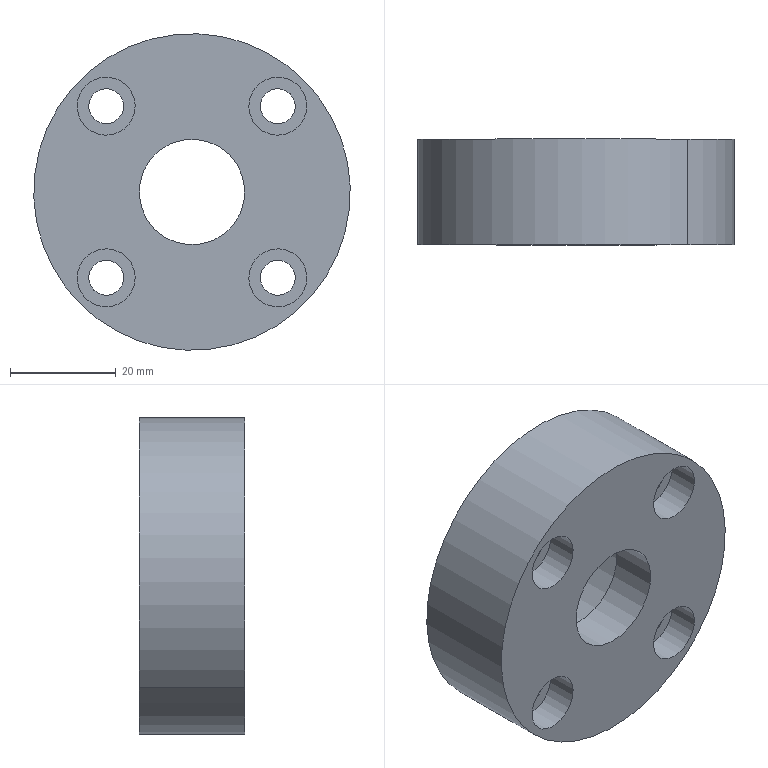Component | SolidWorks | LowerRollerFixingRing-5 | 1 solid | 29 faces | box 60 x 20 x 60 mm | volume 38941 mm3 | cylinder 22 | plane 7 | commonest cylinder face diameters 11 x8 6.6 x8 20 x2 35 x2 60 x2
STEP:
#1=COLOUR_RGB('',0.7922,0.8196,0.9333);
#2=FILL_AREA_STYLE_COLOUR('',#1);
#3=FILL_AREA_STYLE('',(#2));
#4=SURFACE_STYLE_FILL_AREA(#3);
#5=SURFACE_SIDE_STYLE('',(#4));
#6=SURFACE_STYLE_USAGE(.BOTH.,#5);
#7=PRESENTATION_STYLE_ASSIGNMENT((#6));
#8=CARTESIAN_POINT('',(-5.128,20.59,-6.45));
#9=VERTEX_POINT('',#8);
#10=CARTESIAN_POINT('',(-4.822,20.59,-6.144));
#11=VERTEX_POINT('',#10);
#12=CARTESIAN_POINT('',(-4.975,20.59,-6.297));
#13=DIRECTION('',(0.,-1.,-0.));
#14=DIRECTION('',(0.7071,0.,0.7071));
#15=AXIS2_PLACEMENT_3D('',#12,#13,#14);
#16=CIRCLE('',#15,0.2165);
#17=EDGE_CURVE('',#9,#11,#16,.T.);
#18=ORIENTED_EDGE('',*,*,#17,.F.);
#19=CARTESIAN_POINT('',(-5.128,20.354,-6.45));
#20=VERTEX_POINT('',#19);
#21=CARTESIAN_POINT('',(-5.128,20.354,-6.45));
#22=DIRECTION('',(0.,-1.,-0.));
#23=VECTOR('',#22,39.37);
#24=LINE('',#21,#23);
#25=EDGE_CURVE('',#9,#20,#24,.T.);
#26=ORIENTED_EDGE('',*,*,#25,.T.);
#27=CARTESIAN_POINT('',(-4.822,20.354,-6.144));
#28=VERTEX_POINT('',#27);
#29=CARTESIAN_POINT('',(-4.975,20.354,-6.297));
#30=DIRECTION('',(0.,-1.,-0.));
#31=DIRECTION('',(0.7071,0.,0.7071));
#32=AXIS2_PLACEMENT_3D('',#29,#30,#31);
#33=CIRCLE('',#32,0.2165);
#34=EDGE_CURVE('',#20,#28,#33,.T.);
#35=ORIENTED_EDGE('',*,*,#34,.T.);
#36=CARTESIAN_POINT('',(-4.822,20.354,-6.144));
#37=DIRECTION('',(0.,-1.,-0.));
#38=VECTOR('',#37,39.37);
#39=LINE('',#36,#38);
#40=EDGE_CURVE('',#11,#28,#39,.T.);
#41=ORIENTED_EDGE('',*,*,#40,.F.);
#42=EDGE_LOOP('',(#18,#26,#35,#41));
#43=FACE_OUTER_BOUND('',#42,.T.);
#44=CARTESIAN_POINT('',(-4.975,20.354,-6.297));
#45=DIRECTION('',(0.,-1.,-0.));
#46=DIRECTION('',(0.7071,0.,0.7071));
#47=AXIS2_PLACEMENT_3D('',#44,#45,#46);
#48=CYLINDRICAL_SURFACE('',#47,0.2165);
#49=ADVANCED_FACE('',(#43),#48,.F.);
#50=CARTESIAN_POINT('',(-5.067,21.141,-6.389));
#51=VERTEX_POINT('',#50);
#52=CARTESIAN_POINT('',(-4.883,21.141,-6.205));
#53=VERTEX_POINT('',#52);
#54=CARTESIAN_POINT('',(-4.975,21.141,-6.297));
#55=DIRECTION('',(0.,-1.,-0.));
#56=DIRECTION('',(0.7071,0.,0.7071));
#57=AXIS2_PLACEMENT_3D('',#54,#55,#56);
#58=CIRCLE('',#57,0.1299);
#59=EDGE_CURVE('',#51,#53,#58,.T.);
#60=ORIENTED_EDGE('',*,*,#59,.F.);
#61=CARTESIAN_POINT('',(-5.067,20.59,-6.389));
#62=VERTEX_POINT('',#61);
#63=CARTESIAN_POINT('',(-5.067,20.354,-6.389));
#64=DIRECTION('',(0.,-1.,-0.));
#65=VECTOR('',#64,39.37);
#66=LINE('',#63,#65);
#67=EDGE_CURVE('',#51,#62,#66,.T.);
#68=ORIENTED_EDGE('',*,*,#67,.T.);
#69=CARTESIAN_POINT('',(-4.883,20.59,-6.205));
#70=VERTEX_POINT('',#69);
#71=CARTESIAN_POINT('',(-4.975,20.59,-6.297));
#72=DIRECTION('',(0.,-1.,-0.));
#73=DIRECTION('',(0.7071,0.,0.7071));
#74=AXIS2_PLACEMENT_3D('',#71,#72,#73);
#75=CIRCLE('',#74,0.1299);
#76=EDGE_CURVE('',#62,#70,#75,.T.);
#77=ORIENTED_EDGE('',*,*,#76,.T.);
#78=CARTESIAN_POINT('',(-4.883,20.354,-6.205));
#79=DIRECTION('',(0.,-1.,-0.));
#80=VECTOR('',#79,39.37);
#81=LINE('',#78,#80);
#82=EDGE_CURVE('',#53,#70,#81,.T.);
#83=ORIENTED_EDGE('',*,*,#82,.F.);
#84=EDGE_LOOP('',(#60,#68,#77,#83));
#85=FACE_OUTER_BOUND('',#84,.T.);
#86=CARTESIAN_POINT('',(-4.975,20.354,-6.297));
#87=DIRECTION('',(0.,-1.,-0.));
#88=DIRECTION('',(0.7071,0.,0.7071));
#89=AXIS2_PLACEMENT_3D('',#86,#87,#88);
#90=CYLINDRICAL_SURFACE('',#89,0.1299);
#91=ADVANCED_FACE('',(#85),#90,.F.);
#92=CARTESIAN_POINT('',(-5.128,20.59,-7.731));
#93=VERTEX_POINT('',#92);
#94=CARTESIAN_POINT('',(-4.822,20.59,-7.425));
#95=VERTEX_POINT('',#94);
#96=CARTESIAN_POINT('',(-4.975,20.59,-7.578));
#97=DIRECTION('',(0.,-1.,-0.));
#98=DIRECTION('',(0.7071,0.,0.7071));
#99=AXIS2_PLACEMENT_3D('',#96,#97,#98);
#100=CIRCLE('',#99,0.2165);
#101=EDGE_CURVE('',#93,#95,#100,.T.);
#102=ORIENTED_EDGE('',*,*,#101,.F.);
#103=CARTESIAN_POINT('',(-5.128,20.354,-7.731));
#104=VERTEX_POINT('',#103);
#105=CARTESIAN_POINT('',(-5.128,20.354,-7.731));
#106=DIRECTION('',(0.,-1.,-0.));
#107=VECTOR('',#106,39.37);
#108=LINE('',#105,#107);
#109=EDGE_CURVE('',#93,#104,#108,.T.);
#110=ORIENTED_EDGE('',*,*,#109,.T.);
#111=CARTESIAN_POINT('',(-4.822,20.354,-7.425));
#112=VERTEX_POINT('',#111);
#113=CARTESIAN_POINT('',(-4.975,20.354,-7.578));
#114=DIRECTION('',(0.,-1.,-0.));
#115=DIRECTION('',(0.7071,0.,0.7071));
#116=AXIS2_PLACEMENT_3D('',#113,#114,#115);
#117=CIRCLE('',#116,0.2165);
#118=EDGE_CURVE('',#104,#112,#117,.T.);
#119=ORIENTED_EDGE('',*,*,#118,.T.);
#120=CARTESIAN_POINT('',(-4.822,20.354,-7.425));
#121=DIRECTION('',(0.,-1.,-0.));
#122=VECTOR('',#121,39.37);
#123=LINE('',#120,#122);
#124=EDGE_CURVE('',#95,#112,#123,.T.);
#125=ORIENTED_EDGE('',*,*,#124,.F.);
#126=EDGE_LOOP('',(#102,#110,#119,#125));
#127=FACE_OUTER_BOUND('',#126,.T.);
#128=CARTESIAN_POINT('',(-4.975,20.354,-7.578));
#129=DIRECTION('',(0.,-1.,-0.));
#130=DIRECTION('',(0.7071,0.,0.7071));
#131=AXIS2_PLACEMENT_3D('',#128,#129,#130);
#132=CYLINDRICAL_SURFACE('',#131,0.2165);
#133=ADVANCED_FACE('',(#127),#132,.F.);
#134=CARTESIAN_POINT('',(-5.067,21.141,-7.67));
#135=VERTEX_POINT('',#134);
#136=CARTESIAN_POINT('',(-4.883,21.141,-7.486));
#137=VERTEX_POINT('',#136);
#138=CARTESIAN_POINT('',(-4.975,21.141,-7.578));
#139=DIRECTION('',(0.,-1.,-0.));
#140=DIRECTION('',(0.7071,0.,0.7071));
#141=AXIS2_PLACEMENT_3D('',#138,#139,#140);
#142=CIRCLE('',#141,0.1299);
#143=EDGE_CURVE('',#135,#137,#142,.T.);
#144=ORIENTED_EDGE('',*,*,#143,.F.);
#145=CARTESIAN_POINT('',(-5.067,20.59,-7.67));
#146=VERTEX_POINT('',#145);
#147=CARTESIAN_POINT('',(-5.067,20.354,-7.67));
#148=DIRECTION('',(0.,-1.,-0.));
#149=VECTOR('',#148,39.37);
#150=LINE('',#147,#149);
#151=EDGE_CURVE('',#135,#146,#150,.T.);
#152=ORIENTED_EDGE('',*,*,#151,.T.);
#153=CARTESIAN_POINT('',(-4.883,20.59,-7.486));
#154=VERTEX_POINT('',#153);
#155=CARTESIAN_POINT('',(-4.975,20.59,-7.578));
#156=DIRECTION('',(0.,-1.,-0.));
#157=DIRECTION('',(0.7071,0.,0.7071));
#158=AXIS2_PLACEMENT_3D('',#155,#156,#157);
#159=CIRCLE('',#158,0.1299);
#160=EDGE_CURVE('',#146,#154,#159,.T.);
#161=ORIENTED_EDGE('',*,*,#160,.T.);
#162=CARTESIAN_POINT('',(-4.883,20.354,-7.486));
#163=DIRECTION('',(0.,-1.,-0.));
#164=VECTOR('',#163,39.37);
#165=LINE('',#162,#164);
#166=EDGE_CURVE('',#137,#154,#165,.T.);
#167=ORIENTED_EDGE('',*,*,#166,.F.);
#168=EDGE_LOOP('',(#144,#152,#161,#167));
#169=FACE_OUTER_BOUND('',#168,.T.);
#170=CARTESIAN_POINT('',(-4.975,20.354,-7.578));
#171=DIRECTION('',(0.,-1.,-0.));
#172=DIRECTION('',(0.7071,0.,0.7071));
#173=AXIS2_PLACEMENT_3D('',#170,#171,#172);
#174=CYLINDRICAL_SURFACE('',#173,0.1299);
#175=ADVANCED_FACE('',(#169),#174,.F.);
#176=CARTESIAN_POINT('',(-6.408,20.59,-6.45));
#177=VERTEX_POINT('',#176);
#178=CARTESIAN_POINT('',(-6.102,20.59,-6.144));
#179=VERTEX_POINT('',#178);
#180=CARTESIAN_POINT('',(-6.255,20.59,-6.297));
#181=DIRECTION('',(0.,-1.,-0.));
#182=DIRECTION('',(0.7071,0.,0.7071));
#183=AXIS2_PLACEMENT_3D('',#180,#181,#182);
#184=CIRCLE('',#183,0.2165);
#185=EDGE_CURVE('',#177,#179,#184,.T.);
#186=ORIENTED_EDGE('',*,*,#185,.F.);
#187=CARTESIAN_POINT('',(-6.408,20.354,-6.45));
#188=VERTEX_POINT('',#187);
#189=CARTESIAN_POINT('',(-6.408,20.354,-6.45));
#190=DIRECTION('',(0.,-1.,-0.));
#191=VECTOR('',#190,39.37);
#192=LINE('',#189,#191);
#193=EDGE_CURVE('',#177,#188,#192,.T.);
#194=ORIENTED_EDGE('',*,*,#193,.T.);
#195=CARTESIAN_POINT('',(-6.102,20.354,-6.144));
#196=VERTEX_POINT('',#195);
#197=CARTESIAN_POINT('',(-6.255,20.354,-6.297));
#198=DIRECTION('',(0.,-1.,-0.));
#199=DIRECTION('',(0.7071,0.,0.7071));
#200=AXIS2_PLACEMENT_3D('',#197,#198,#199);
#201=CIRCLE('',#200,0.2165);
#202=EDGE_CURVE('',#188,#196,#201,.T.);
#203=ORIENTED_EDGE('',*,*,#202,.T.);
#204=CARTESIAN_POINT('',(-6.102,20.354,-6.144));
#205=DIRECTION('',(0.,-1.,-0.));
#206=VECTOR('',#205,39.37);
#207=LINE('',#204,#206);
#208=EDGE_CURVE('',#179,#196,#207,.T.);
#209=ORIENTED_EDGE('',*,*,#208,.F.);
#210=EDGE_LOOP('',(#186,#194,#203,#209));
#211=FACE_OUTER_BOUND('',#210,.T.);
#212=CARTESIAN_POINT('',(-6.255,20.354,-6.297));
#213=DIRECTION('',(0.,-1.,-0.));
#214=DIRECTION('',(0.7071,0.,0.7071));
#215=AXIS2_PLACEMENT_3D('',#212,#213,#214);
#216=CYLINDRICAL_SURFACE('',#215,0.2165);
#217=ADVANCED_FACE('',(#211),#216,.F.);
#218=CARTESIAN_POINT('',(-6.347,21.141,-6.389));
#219=VERTEX_POINT('',#218);
#220=CARTESIAN_POINT('',(-6.163,21.141,-6.205));
#221=VERTEX_POINT('',#220);
#222=CARTESIAN_POINT('',(-6.255,21.141,-6.297));
#223=DIRECTION('',(0.,-1.,-0.));
#224=DIRECTION('',(0.7071,0.,0.7071));
#225=AXIS2_PLACEMENT_3D('',#222,#223,#224);
#226=CIRCLE('',#225,0.1299);
#227=EDGE_CURVE('',#219,#221,#226,.T.);
#228=ORIENTED_EDGE('',*,*,#227,.F.);
#229=CARTESIAN_POINT('',(-6.347,20.59,-6.389));
#230=VERTEX_POINT('',#229);
#231=CARTESIAN_POINT('',(-6.347,20.354,-6.389));
#232=DIRECTION('',(0.,-1.,-0.));
#233=VECTOR('',#232,39.37);
#234=LINE('',#231,#233);
#235=EDGE_CURVE('',#219,#230,#234,.T.);
#236=ORIENTED_EDGE('',*,*,#235,.T.);
#237=CARTESIAN_POINT('',(-6.163,20.59,-6.205));
#238=VERTEX_POINT('',#237);
#239=CARTESIAN_POINT('',(-6.255,20.59,-6.297));
#240=DIRECTION('',(0.,-1.,-0.));
#241=DIRECTION('',(0.7071,0.,0.7071));
#242=AXIS2_PLACEMENT_3D('',#239,#240,#241);
#243=CIRCLE('',#242,0.1299);
#244=EDGE_CURVE('',#230,#238,#243,.T.);
#245=ORIENTED_EDGE('',*,*,#244,.T.);
#246=CARTESIAN_POINT('',(-6.163,20.354,-6.205));
#247=DIRECTION('',(0.,-1.,-0.));
#248=VECTOR('',#247,39.37);
#249=LINE('',#246,#248);
#250=EDGE_CURVE('',#221,#238,#249,.T.);
#251=ORIENTED_EDGE('',*,*,#250,.F.);
#252=EDGE_LOOP('',(#228,#236,#245,#251));
#253=FACE_OUTER_BOUND('',#252,.T.);
#254=CARTESIAN_POINT('',(-6.255,20.354,-6.297));
#255=DIRECTION('',(0.,-1.,-0.));
#256=DIRECTION('',(0.7071,0.,0.7071));
#257=AXIS2_PLACEMENT_3D('',#254,#255,#256);
#258=CYLINDRICAL_SURFACE('',#257,0.1299);
#259=ADVANCED_FACE('',(#253),#258,.F.);
#260=CARTESIAN_POINT('',(-6.408,20.59,-7.731));
#261=VERTEX_POINT('',#260);
#262=CARTESIAN_POINT('',(-6.102,20.59,-7.425));
#263=VERTEX_POINT('',#262);
#264=CARTESIAN_POINT('',(-6.255,20.59,-7.578));
#265=DIRECTION('',(0.,-1.,-0.));
#266=DIRECTION('',(0.7071,0.,0.7071));
#267=AXIS2_PLACEMENT_3D('',#264,#265,#266);
#268=CIRCLE('',#267,0.2165);
#269=EDGE_CURVE('',#261,#263,#268,.T.);
#270=ORIENTED_EDGE('',*,*,#269,.F.);
#271=CARTESIAN_POINT('',(-6.408,20.354,-7.731));
#272=VERTEX_POINT('',#271);
#273=CARTESIAN_POINT('',(-6.408,20.354,-7.731));
#274=DIRECTION('',(0.,-1.,-0.));
#275=VECTOR('',#274,39.37);
#276=LINE('',#273,#275);
#277=EDGE_CURVE('',#261,#272,#276,.T.);
#278=ORIENTED_EDGE('',*,*,#277,.T.);
#279=CARTESIAN_POINT('',(-6.102,20.354,-7.425));
#280=VERTEX_POINT('',#279);
#281=CARTESIAN_POINT('',(-6.255,20.354,-7.578));
#282=DIRECTION('',(0.,-1.,-0.));
#283=DIRECTION('',(0.7071,0.,0.7071));
#284=AXIS2_PLACEMENT_3D('',#281,#282,#283);
#285=CIRCLE('',#284,0.2165);
#286=EDGE_CURVE('',#272,#280,#285,.T.);
#287=ORIENTED_EDGE('',*,*,#286,.T.);
#288=CARTESIAN_POINT('',(-6.102,20.354,-7.425));
#289=DIRECTION('',(0.,-1.,-0.));
#290=VECTOR('',#289,39.37);
#291=LINE('',#288,#290);
#292=EDGE_CURVE('',#263,#280,#291,.T.);
#293=ORIENTED_EDGE('',*,*,#292,.F.);
#294=EDGE_LOOP('',(#270,#278,#287,#293));
#295=FACE_OUTER_BOUND('',#294,.T.);
#296=CARTESIAN_POINT('',(-6.255,20.354,-7.578));
#297=DIRECTION('',(0.,-1.,-0.));
#298=DIRECTION('',(0.7071,0.,0.7071));
#299=AXIS2_PLACEMENT_3D('',#296,#297,#298);
#300=CYLINDRICAL_SURFACE('',#299,0.2165);
#301=ADVANCED_FACE('',(#295),#300,.F.);
#302=CARTESIAN_POINT('',(-6.347,21.141,-7.67));
#303=VERTEX_POINT('',#302);
#304=CARTESIAN_POINT('',(-6.163,21.141,-7.486));
#305=VERTEX_POINT('',#304);
#306=CARTESIAN_POINT('',(-6.255,21.141,-7.578));
#307=DIRECTION('',(0.,-1.,-0.));
#308=DIRECTION('',(0.7071,0.,0.7071));
#309=AXIS2_PLACEMENT_3D('',#306,#307,#308);
#310=CIRCLE('',#309,0.1299);
#311=EDGE_CURVE('',#303,#305,#310,.T.);
#312=ORIENTED_EDGE('',*,*,#311,.F.);
#313=CARTESIAN_POINT('',(-6.347,20.59,-7.67));
#314=VERTEX_POINT('',#313);
#315=CARTESIAN_POINT('',(-6.347,20.354,-7.67));
#316=DIRECTION('',(0.,-1.,-0.));
#317=VECTOR('',#316,39.37);
#318=LINE('',#315,#317);
#319=EDGE_CURVE('',#303,#314,#318,.T.);
#320=ORIENTED_EDGE('',*,*,#319,.T.);
#321=CARTESIAN_POINT('',(-6.163,20.59,-7.486));
#322=VERTEX_POINT('',#321);
#323=CARTESIAN_POINT('',(-6.255,20.59,-7.578));
#324=DIRECTION('',(0.,-1.,-0.));
#325=DIRECTION('',(0.7071,0.,0.7071));
#326=AXIS2_PLACEMENT_3D('',#323,#324,#325);
#327=CIRCLE('',#326,0.1299);
#328=EDGE_CURVE('',#314,#322,#327,.T.);
#329=ORIENTED_EDGE('',*,*,#328,.T.);
#330=CARTESIAN_POINT('',(-6.163,20.354,-7.486));
#331=DIRECTION('',(0.,-1.,-0.));
#332=VECTOR('',#331,39.37);
#333=LINE('',#330,#332);
#334=EDGE_CURVE('',#305,#322,#333,.T.);
#335=ORIENTED_EDGE('',*,*,#334,.F.);
#336=EDGE_LOOP('',(#312,#320,#329,#335));
#337=FACE_OUTER_BOUND('',#336,.T.);
#338=CARTESIAN_POINT('',(-6.255,20.354,-7.578));
#339=DIRECTION('',(0.,-1.,-0.));
#340=DIRECTION('',(0.7071,0.,0.7071));
#341=AXIS2_PLACEMENT_3D('',#338,#339,#340);
#342=CYLINDRICAL_SURFACE('',#341,0.1299);
#343=ADVANCED_FACE('',(#337),#342,.F.);
#344=CARTESIAN_POINT('',(-5.337,20.354,-6.659));
#345=VERTEX_POINT('',#344);
#346=CARTESIAN_POINT('',(-5.893,20.354,-7.216));
#347=VERTEX_POINT('',#346);
#348=CARTESIAN_POINT('',(-5.615,20.354,-6.938));
#349=DIRECTION('',(-0.,1.,0.));
#350=DIRECTION('',(-0.7071,0.,-0.7071));
#351=AXIS2_PLACEMENT_3D('',#348,#349,#350);
#352=CIRCLE('',#351,0.3937);
#353=EDGE_CURVE('',#345,#347,#352,.T.);
#354=ORIENTED_EDGE('',*,*,#353,.F.);
#355=CARTESIAN_POINT('',(-5.337,20.708,-6.659));
#356=VERTEX_POINT('',#355);
#357=CARTESIAN_POINT('',(-5.337,21.359,-6.659));
#358=DIRECTION('',(-0.,1.,0.));
#359=VECTOR('',#358,39.37);
#360=LINE('',#357,#359);
#361=EDGE_CURVE('',#345,#356,#360,.T.);
#362=ORIENTED_EDGE('',*,*,#361,.T.);
#363=CARTESIAN_POINT('',(-5.893,20.708,-7.216));
#364=VERTEX_POINT('',#363);
#365=CARTESIAN_POINT('',(-5.615,20.708,-6.938));
#366=DIRECTION('',(-0.,1.,0.));
#367=DIRECTION('',(-0.7071,0.,-0.7071));
#368=AXIS2_PLACEMENT_3D('',#365,#366,#367);
#369=CIRCLE('',#368,0.3937);
#370=EDGE_CURVE('',#356,#364,#369,.T.);
#371=ORIENTED_EDGE('',*,*,#370,.T.);
#372=CARTESIAN_POINT('',(-5.893,21.359,-7.216));
#373=DIRECTION('',(-0.,1.,0.));
#374=VECTOR('',#373,39.37);
#375=LINE('',#372,#374);
#376=EDGE_CURVE('',#347,#364,#375,.T.);
#377=ORIENTED_EDGE('',*,*,#376,.F.);
#378=EDGE_LOOP('',(#354,#362,#371,#377));
#379=FACE_OUTER_BOUND('',#378,.T.);
#380=CARTESIAN_POINT('',(-5.615,21.359,-6.938));
#381=DIRECTION('',(-0.,1.,0.));
#382=DIRECTION('',(-0.7071,0.,-0.7071));
#383=AXIS2_PLACEMENT_3D('',#380,#381,#382);
#384=CYLINDRICAL_SURFACE('',#383,0.3937);
#385=ADVANCED_FACE('',(#379),#384,.F.);
#386=CARTESIAN_POINT('',(-5.128,20.708,-6.45));
#387=VERTEX_POINT('',#386);
#388=CARTESIAN_POINT('',(-6.102,20.708,-7.425));
#389=VERTEX_POINT('',#388);
#390=CARTESIAN_POINT('',(-5.615,20.708,-6.938));
#391=DIRECTION('',(-0.,1.,0.));
#392=DIRECTION('',(-0.7071,0.,-0.7071));
#393=AXIS2_PLACEMENT_3D('',#390,#391,#392);
#394=CIRCLE('',#393,0.689);
#395=EDGE_CURVE('',#387,#389,#394,.T.);
#396=ORIENTED_EDGE('',*,*,#395,.F.);
#397=CARTESIAN_POINT('',(-5.128,21.141,-6.45));
#398=VERTEX_POINT('',#397);
#399=CARTESIAN_POINT('',(-5.128,21.359,-6.45));
#400=DIRECTION('',(-0.,1.,0.));
#401=VECTOR('',#400,39.37);
#402=LINE('',#399,#401);
#403=EDGE_CURVE('',#387,#398,#402,.T.);
#404=ORIENTED_EDGE('',*,*,#403,.T.);
#405=CARTESIAN_POINT('',(-6.102,21.141,-7.425));
#406=VERTEX_POINT('',#405);
#407=CARTESIAN_POINT('',(-5.615,21.141,-6.938));
#408=DIRECTION('',(-0.,1.,0.));
#409=DIRECTION('',(-0.7071,0.,-0.7071));
#410=AXIS2_PLACEMENT_3D('',#407,#408,#409);
#411=CIRCLE('',#410,0.689);
#412=EDGE_CURVE('',#398,#406,#411,.T.);
#413=ORIENTED_EDGE('',*,*,#412,.T.);
#414=CARTESIAN_POINT('',(-6.102,21.359,-7.425));
#415=DIRECTION('',(-0.,1.,0.));
#416=VECTOR('',#415,39.37);
#417=LINE('',#414,#416);
#418=EDGE_CURVE('',#389,#406,#417,.T.);
#419=ORIENTED_EDGE('',*,*,#418,.F.);
#420=EDGE_LOOP('',(#396,#404,#413,#419));
#421=FACE_OUTER_BOUND('',#420,.T.);
#422=CARTESIAN_POINT('',(-5.615,21.359,-6.938));
#423=DIRECTION('',(-0.,1.,0.));
#424=DIRECTION('',(-0.7071,0.,-0.7071));
#425=AXIS2_PLACEMENT_3D('',#422,#423,#424);
#426=CYLINDRICAL_SURFACE('',#425,0.689);
#427=ADVANCED_FACE('',(#421),#426,.F.);
#428=CARTESIAN_POINT('',(-6.45,20.354,-7.773));
#429=VERTEX_POINT('',#428);
#430=CARTESIAN_POINT('',(-4.78,20.354,-6.102));
#431=VERTEX_POINT('',#430);
#432=CARTESIAN_POINT('',(-5.615,20.354,-6.938));
#433=DIRECTION('',(-0.,1.,0.));
#434=DIRECTION('',(-0.7071,0.,-0.7071));
#435=AXIS2_PLACEMENT_3D('',#432,#433,#434);
#436=CIRCLE('',#435,1.181);
#437=EDGE_CURVE('',#429,#431,#436,.T.);
#438=ORIENTED_EDGE('',*,*,#437,.T.);
#439=CARTESIAN_POINT('',(-4.78,21.141,-6.102));
#440=VERTEX_POINT('',#439);
#441=CARTESIAN_POINT('',(-4.78,21.359,-6.102));
#442=DIRECTION('',(-0.,1.,0.));
#443=VECTOR('',#442,39.37);
#444=LINE('',#441,#443);
#445=EDGE_CURVE('',#431,#440,#444,.T.);
#446=ORIENTED_EDGE('',*,*,#445,.T.);
#447=CARTESIAN_POINT('',(-6.45,21.141,-7.773));
#448=VERTEX_POINT('',#447);
#449=CARTESIAN_POINT('',(-5.615,21.141,-6.938));
#450=DIRECTION('',(-0.,1.,0.));
#451=DIRECTION('',(-0.7071,0.,-0.7071));
#452=AXIS2_PLACEMENT_3D('',#449,#450,#451);
#453=CIRCLE('',#452,1.181);
#454=EDGE_CURVE('',#448,#440,#453,.T.);
#455=ORIENTED_EDGE('',*,*,#454,.F.);
#456=CARTESIAN_POINT('',(-6.45,21.359,-7.773));
#457=DIRECTION('',(-0.,1.,0.));
#458=VECTOR('',#457,39.37);
#459=LINE('',#456,#458);
#460=EDGE_CURVE('',#429,#448,#459,.T.);
#461=ORIENTED_EDGE('',*,*,#460,.F.);
#462=EDGE_LOOP('',(#438,#446,#455,#461));
#463=FACE_OUTER_BOUND('',#462,.T.);
#464=CARTESIAN_POINT('',(-5.615,21.359,-6.938));
#465=DIRECTION('',(-0.,1.,0.));
#466=DIRECTION('',(-0.7071,0.,-0.7071));
#467=AXIS2_PLACEMENT_3D('',#464,#465,#466);
#468=CYLINDRICAL_SURFACE('',#467,1.181);
#469=ADVANCED_FACE('',(#463),#468,.T.);
#470=ORIENTED_EDGE('',*,*,#445,.F.);
#471=CARTESIAN_POINT('',(-5.615,20.354,-6.938));
#472=DIRECTION('',(-0.,1.,0.));
#473=DIRECTION('',(-0.7071,0.,-0.7071));
#474=AXIS2_PLACEMENT_3D('',#471,#472,#473);
#475=CIRCLE('',#474,1.181);
#476=EDGE_CURVE('',#431,#429,#475,.T.);
#477=ORIENTED_EDGE('',*,*,#476,.T.);
#478=ORIENTED_EDGE('',*,*,#460,.T.);
#479=CARTESIAN_POINT('',(-5.615,21.141,-6.938));
#480=DIRECTION('',(-0.,1.,0.));
#481=DIRECTION('',(-0.7071,0.,-0.7071));
#482=AXIS2_PLACEMENT_3D('',#479,#480,#481);
#483=CIRCLE('',#482,1.181);
#484=EDGE_CURVE('',#440,#448,#483,.T.);
#485=ORIENTED_EDGE('',*,*,#484,.F.);
#486=EDGE_LOOP('',(#470,#477,#478,#485));
#487=FACE_OUTER_BOUND('',#486,.T.);
#488=CARTESIAN_POINT('',(-5.615,21.359,-6.938));
#489=DIRECTION('',(-0.,1.,0.));
#490=DIRECTION('',(-0.7071,0.,-0.7071));
#491=AXIS2_PLACEMENT_3D('',#488,#489,#490);
#492=CYLINDRICAL_SURFACE('',#491,1.181);
#493=ADVANCED_FACE('',(#487),#492,.T.);
#494=CARTESIAN_POINT('',(-4.975,21.141,-6.297));
#495=DIRECTION('',(0.,-1.,-0.));
#496=DIRECTION('',(0.7071,0.,0.7071));
#497=AXIS2_PLACEMENT_3D('',#494,#495,#496);
#498=CIRCLE('',#497,0.1299);
#499=EDGE_CURVE('',#53,#51,#498,.T.);
#500=ORIENTED_EDGE('',*,*,#499,.T.);
#501=ORIENTED_EDGE('',*,*,#59,.T.);
#502=EDGE_LOOP('',(#500,#501));
#503=FACE_BOUND('',#502,.T.);
#504=CARTESIAN_POINT('',(-4.975,21.141,-7.578));
#505=DIRECTION('',(0.,-1.,-0.));
#506=DIRECTION('',(0.7071,0.,0.7071));
#507=AXIS2_PLACEMENT_3D('',#504,#505,#506);
#508=CIRCLE('',#507,0.1299);
#509=EDGE_CURVE('',#137,#135,#508,.T.);
#510=ORIENTED_EDGE('',*,*,#509,.T.);
#511=ORIENTED_EDGE('',*,*,#143,.T.);
#512=EDGE_LOOP('',(#510,#511));
#513=FACE_BOUND('',#512,.T.);
#514=CARTESIAN_POINT('',(-6.255,21.141,-6.297));
#515=DIRECTION('',(0.,-1.,-0.));
#516=DIRECTION('',(0.7071,0.,0.7071));
#517=AXIS2_PLACEMENT_3D('',#514,#515,#516);
#518=CIRCLE('',#517,0.1299);
#519=EDGE_CURVE('',#221,#219,#518,.T.);
#520=ORIENTED_EDGE('',*,*,#519,.T.);
#521=ORIENTED_EDGE('',*,*,#227,.T.);
#522=EDGE_LOOP('',(#520,#521));
#523=FACE_BOUND('',#522,.T.);
#524=CARTESIAN_POINT('',(-6.255,21.141,-7.578));
#525=DIRECTION('',(0.,-1.,-0.));
#526=DIRECTION('',(0.7071,0.,0.7071));
#527=AXIS2_PLACEMENT_3D('',#524,#525,#526);
#528=CIRCLE('',#527,0.1299);
#529=EDGE_CURVE('',#305,#303,#528,.T.);
#530=ORIENTED_EDGE('',*,*,#529,.T.);
#531=ORIENTED_EDGE('',*,*,#311,.T.);
#532=EDGE_LOOP('',(#530,#531));
#533=FACE_BOUND('',#532,.T.);
#534=ORIENTED_EDGE('',*,*,#454,.T.);
#535=ORIENTED_EDGE('',*,*,#484,.T.);
#536=EDGE_LOOP('',(#534,#535));
#537=FACE_OUTER_BOUND('',#536,.T.);
#538=CARTESIAN_POINT('',(-5.615,21.141,-6.938));
#539=DIRECTION('',(-0.,1.,0.));
#540=DIRECTION('',(-0.7071,0.,-0.7071));
#541=AXIS2_PLACEMENT_3D('',#538,#539,#540);
#542=CIRCLE('',#541,0.689);
#543=EDGE_CURVE('',#406,#398,#542,.T.);
#544=ORIENTED_EDGE('',*,*,#543,.F.);
#545=ORIENTED_EDGE('',*,*,#412,.F.);
#546=EDGE_LOOP('',(#544,#545));
#547=FACE_BOUND('',#546,.T.);
#548=CARTESIAN_POINT('',(-6.45,21.141,-6.102));
#549=DIRECTION('',(-0.,1.,0.));
#550=DIRECTION('',(-0.7071,0.,-0.7071));
#551=AXIS2_PLACEMENT_3D('',#548,#549,#550);
#552=PLANE('',#551);
#553=ADVANCED_FACE('',(#503,#513,#523,#533,#537,#547),#552,.T.);
#554=ORIENTED_EDGE('',*,*,#403,.F.);
#555=CARTESIAN_POINT('',(-5.615,20.708,-6.938));
#556=DIRECTION('',(-0.,1.,0.));
#557=DIRECTION('',(-0.7071,0.,-0.7071));
#558=AXIS2_PLACEMENT_3D('',#555,#556,#557);
#559=CIRCLE('',#558,0.689);
#560=EDGE_CURVE('',#389,#387,#559,.T.);
#561=ORIENTED_EDGE('',*,*,#560,.F.);
#562=ORIENTED_EDGE('',*,*,#418,.T.);
#563=ORIENTED_EDGE('',*,*,#543,.T.);
#564=EDGE_LOOP('',(#554,#561,#562,#563));
#565=FACE_OUTER_BOUND('',#564,.T.);
#566=CARTESIAN_POINT('',(-5.615,21.359,-6.938));
#567=DIRECTION('',(-0.,1.,0.));
#568=DIRECTION('',(-0.7071,0.,-0.7071));
#569=AXIS2_PLACEMENT_3D('',#566,#567,#568);
#570=CYLINDRICAL_SURFACE('',#569,0.689);
#571=ADVANCED_FACE('',(#565),#570,.F.);
#572=ORIENTED_EDGE('',*,*,#560,.T.);
#573=ORIENTED_EDGE('',*,*,#395,.T.);
#574=EDGE_LOOP('',(#572,#573));
#575=FACE_OUTER_BOUND('',#574,.T.);
#576=CARTESIAN_POINT('',(-5.615,20.708,-6.938));
#577=DIRECTION('',(-0.,1.,0.));
#578=DIRECTION('',(-0.7071,0.,-0.7071));
#579=AXIS2_PLACEMENT_3D('',#576,#577,#578);
#580=CIRCLE('',#579,0.3937);
#581=EDGE_CURVE('',#364,#356,#580,.T.);
#582=ORIENTED_EDGE('',*,*,#581,.F.);
#583=ORIENTED_EDGE('',*,*,#370,.F.);
#584=EDGE_LOOP('',(#582,#583));
#585=FACE_BOUND('',#584,.T.);
#586=CARTESIAN_POINT('',(-6.102,20.708,-6.45));
#587=DIRECTION('',(-0.,1.,0.));
#588=DIRECTION('',(-0.7071,0.,-0.7071));
#589=AXIS2_PLACEMENT_3D('',#586,#587,#588);
#590=PLANE('',#589);
#591=ADVANCED_FACE('',(#575,#585),#590,.T.);
#592=ORIENTED_EDGE('',*,*,#361,.F.);
#593=CARTESIAN_POINT('',(-5.615,20.354,-6.938));
#594=DIRECTION('',(-0.,1.,0.));
#595=DIRECTION('',(-0.7071,0.,-0.7071));
#596=AXIS2_PLACEMENT_3D('',#593,#594,#595);
#597=CIRCLE('',#596,0.3937);
#598=EDGE_CURVE('',#347,#345,#597,.T.);
#599=ORIENTED_EDGE('',*,*,#598,.F.);
#600=ORIENTED_EDGE('',*,*,#376,.T.);
#601=ORIENTED_EDGE('',*,*,#581,.T.);
#602=EDGE_LOOP('',(#592,#599,#600,#601));
#603=FACE_OUTER_BOUND('',#602,.T.);
#604=CARTESIAN_POINT('',(-5.615,21.359,-6.938));
#605=DIRECTION('',(-0.,1.,0.));
#606=DIRECTION('',(-0.7071,0.,-0.7071));
#607=AXIS2_PLACEMENT_3D('',#604,#605,#606);
#608=CYLINDRICAL_SURFACE('',#607,0.3937);
#609=ADVANCED_FACE('',(#603),#608,.F.);
#610=CARTESIAN_POINT('',(-4.975,20.354,-6.297));
#611=DIRECTION('',(0.,-1.,-0.));
#612=DIRECTION('',(0.7071,0.,0.7071));
#613=AXIS2_PLACEMENT_3D('',#610,#611,#612);
#614=CIRCLE('',#613,0.2165);
#615=EDGE_CURVE('',#28,#20,#614,.T.);
#616=ORIENTED_EDGE('',*,*,#615,.F.);
#617=ORIENTED_EDGE('',*,*,#34,.F.);
#618=EDGE_LOOP('',(#616,#617));
#619=FACE_BOUND('',#618,.T.);
#620=CARTESIAN_POINT('',(-4.975,20.354,-7.578));
#621=DIRECTION('',(0.,-1.,-0.));
#622=DIRECTION('',(0.7071,0.,0.7071));
#623=AXIS2_PLACEMENT_3D('',#620,#621,#622);
#624=CIRCLE('',#623,0.2165);
#625=EDGE_CURVE('',#112,#104,#624,.T.);
#626=ORIENTED_EDGE('',*,*,#625,.F.);
#627=ORIENTED_EDGE('',*,*,#118,.F.);
#628=EDGE_LOOP('',(#626,#627));
#629=FACE_BOUND('',#628,.T.);
#630=CARTESIAN_POINT('',(-6.255,20.354,-6.297));
#631=DIRECTION('',(0.,-1.,-0.));
#632=DIRECTION('',(0.7071,0.,0.7071));
#633=AXIS2_PLACEMENT_3D('',#630,#631,#632);
#634=CIRCLE('',#633,0.2165);
#635=EDGE_CURVE('',#196,#188,#634,.T.);
#636=ORIENTED_EDGE('',*,*,#635,.F.);
#637=ORIENTED_EDGE('',*,*,#202,.F.);
#638=EDGE_LOOP('',(#636,#637));
#639=FACE_BOUND('',#638,.T.);
#640=CARTESIAN_POINT('',(-6.255,20.354,-7.578));
#641=DIRECTION('',(0.,-1.,-0.));
#642=DIRECTION('',(0.7071,0.,0.7071));
#643=AXIS2_PLACEMENT_3D('',#640,#641,#642);
#644=CIRCLE('',#643,0.2165);
#645=EDGE_CURVE('',#280,#272,#644,.T.);
#646=ORIENTED_EDGE('',*,*,#645,.F.);
#647=ORIENTED_EDGE('',*,*,#286,.F.);
#648=EDGE_LOOP('',(#646,#647));
#649=FACE_BOUND('',#648,.T.);
#650=ORIENTED_EDGE('',*,*,#598,.T.);
#651=ORIENTED_EDGE('',*,*,#353,.T.);
#652=EDGE_LOOP('',(#650,#651));
#653=FACE_BOUND('',#652,.T.);
#654=ORIENTED_EDGE('',*,*,#437,.F.);
#655=ORIENTED_EDGE('',*,*,#476,.F.);
#656=EDGE_LOOP('',(#654,#655));
#657=FACE_OUTER_BOUND('',#656,.T.);
#658=CARTESIAN_POINT('',(-5.893,20.354,-6.659));
#659=DIRECTION('',(0.,-1.,-0.));
#660=DIRECTION('',(0.7071,-0.,0.7071));
#661=AXIS2_PLACEMENT_3D('',#658,#659,#660);
#662=PLANE('',#661);
#663=ADVANCED_FACE('',(#619,#629,#639,#649,#653,#657),#662,.T.);
#664=ORIENTED_EDGE('',*,*,#319,.F.);
#665=ORIENTED_EDGE('',*,*,#529,.F.);
#666=ORIENTED_EDGE('',*,*,#334,.T.);
#667=CARTESIAN_POINT('',(-6.255,20.59,-7.578));
#668=DIRECTION('',(0.,-1.,-0.));
#669=DIRECTION('',(0.7071,0.,0.7071));
#670=AXIS2_PLACEMENT_3D('',#667,#668,#669);
#671=CIRCLE('',#670,0.1299);
#672=EDGE_CURVE('',#322,#314,#671,.T.);
#673=ORIENTED_EDGE('',*,*,#672,.T.);
#674=EDGE_LOOP('',(#664,#665,#666,#673));
#675=FACE_OUTER_BOUND('',#674,.T.);
#676=CARTESIAN_POINT('',(-6.255,20.354,-7.578));
#677=DIRECTION('',(0.,-1.,-0.));
#678=DIRECTION('',(0.7071,0.,0.7071));
#679=AXIS2_PLACEMENT_3D('',#676,#677,#678);
#680=CYLINDRICAL_SURFACE('',#679,0.1299);
#681=ADVANCED_FACE('',(#675),#680,.F.);
#682=ORIENTED_EDGE('',*,*,#672,.F.);
#683=ORIENTED_EDGE('',*,*,#328,.F.);
#684=EDGE_LOOP('',(#682,#683));
#685=FACE_BOUND('',#684,.T.);
#686=CARTESIAN_POINT('',(-6.255,20.59,-7.578));
#687=DIRECTION('',(0.,-1.,-0.));
#688=DIRECTION('',(0.7071,0.,0.7071));
#689=AXIS2_PLACEMENT_3D('',#686,#687,#688);
#690=CIRCLE('',#689,0.2165);
#691=EDGE_CURVE('',#263,#261,#690,.T.);
#692=ORIENTED_EDGE('',*,*,#691,.T.);
#693=ORIENTED_EDGE('',*,*,#269,.T.);
#694=EDGE_LOOP('',(#692,#693));
#695=FACE_OUTER_BOUND('',#694,.T.);
#696=CARTESIAN_POINT('',(-6.347,20.59,-7.486));
#697=DIRECTION('',(-0.,1.,0.));
#698=DIRECTION('',(-0.7071,0.,-0.7071));
#699=AXIS2_PLACEMENT_3D('',#696,#697,#698);
#700=PLANE('',#699);
#701=ADVANCED_FACE('',(#685,#695),#700,.F.);
#702=ORIENTED_EDGE('',*,*,#277,.F.);
#703=ORIENTED_EDGE('',*,*,#691,.F.);
#704=ORIENTED_EDGE('',*,*,#292,.T.);
#705=ORIENTED_EDGE('',*,*,#645,.T.);
#706=EDGE_LOOP('',(#702,#703,#704,#705));
#707=FACE_OUTER_BOUND('',#706,.T.);
#708=CARTESIAN_POINT('',(-6.255,20.354,-7.578));
#709=DIRECTION('',(0.,-1.,-0.));
#710=DIRECTION('',(0.7071,0.,0.7071));
#711=AXIS2_PLACEMENT_3D('',#708,#709,#710);
#712=CYLINDRICAL_SURFACE('',#711,0.2165);
#713=ADVANCED_FACE('',(#707),#712,.F.);
#714=ORIENTED_EDGE('',*,*,#235,.F.);
#715=ORIENTED_EDGE('',*,*,#519,.F.);
#716=ORIENTED_EDGE('',*,*,#250,.T.);
#717=CARTESIAN_POINT('',(-6.255,20.59,-6.297));
#718=DIRECTION('',(0.,-1.,-0.));
#719=DIRECTION('',(0.7071,0.,0.7071));
#720=AXIS2_PLACEMENT_3D('',#717,#718,#719);
#721=CIRCLE('',#720,0.1299);
#722=EDGE_CURVE('',#238,#230,#721,.T.);
#723=ORIENTED_EDGE('',*,*,#722,.T.);
#724=EDGE_LOOP('',(#714,#715,#716,#723));
#725=FACE_OUTER_BOUND('',#724,.T.);
#726=CARTESIAN_POINT('',(-6.255,20.354,-6.297));
#727=DIRECTION('',(0.,-1.,-0.));
#728=DIRECTION('',(0.7071,0.,0.7071));
#729=AXIS2_PLACEMENT_3D('',#726,#727,#728);
#730=CYLINDRICAL_SURFACE('',#729,0.1299);
#731=ADVANCED_FACE('',(#725),#730,.F.);
#732=ORIENTED_EDGE('',*,*,#722,.F.);
#733=ORIENTED_EDGE('',*,*,#244,.F.);
#734=EDGE_LOOP('',(#732,#733));
#735=FACE_BOUND('',#734,.T.);
#736=CARTESIAN_POINT('',(-6.255,20.59,-6.297));
#737=DIRECTION('',(0.,-1.,-0.));
#738=DIRECTION('',(0.7071,0.,0.7071));
#739=AXIS2_PLACEMENT_3D('',#736,#737,#738);
#740=CIRCLE('',#739,0.2165);
#741=EDGE_CURVE('',#179,#177,#740,.T.);
#742=ORIENTED_EDGE('',*,*,#741,.T.);
#743=ORIENTED_EDGE('',*,*,#185,.T.);
#744=EDGE_LOOP('',(#742,#743));
#745=FACE_OUTER_BOUND('',#744,.T.);
#746=CARTESIAN_POINT('',(-6.347,20.59,-6.205));
#747=DIRECTION('',(-0.,1.,0.));
#748=DIRECTION('',(-0.7071,0.,-0.7071));
#749=AXIS2_PLACEMENT_3D('',#746,#747,#748);
#750=PLANE('',#749);
#751=ADVANCED_FACE('',(#735,#745),#750,.F.);
#752=ORIENTED_EDGE('',*,*,#193,.F.);
#753=ORIENTED_EDGE('',*,*,#741,.F.);
#754=ORIENTED_EDGE('',*,*,#208,.T.);
#755=ORIENTED_EDGE('',*,*,#635,.T.);
#756=EDGE_LOOP('',(#752,#753,#754,#755));
#757=FACE_OUTER_BOUND('',#756,.T.);
#758=CARTESIAN_POINT('',(-6.255,20.354,-6.297));
#759=DIRECTION('',(0.,-1.,-0.));
#760=DIRECTION('',(0.7071,0.,0.7071));
#761=AXIS2_PLACEMENT_3D('',#758,#759,#760);
#762=CYLINDRICAL_SURFACE('',#761,0.2165);
#763=ADVANCED_FACE('',(#757),#762,.F.);
#764=ORIENTED_EDGE('',*,*,#151,.F.);
#765=ORIENTED_EDGE('',*,*,#509,.F.);
#766=ORIENTED_EDGE('',*,*,#166,.T.);
#767=CARTESIAN_POINT('',(-4.975,20.59,-7.578));
#768=DIRECTION('',(0.,-1.,-0.));
#769=DIRECTION('',(0.7071,0.,0.7071));
#770=AXIS2_PLACEMENT_3D('',#767,#768,#769);
#771=CIRCLE('',#770,0.1299);
#772=EDGE_CURVE('',#154,#146,#771,.T.);
#773=ORIENTED_EDGE('',*,*,#772,.T.);
#774=EDGE_LOOP('',(#764,#765,#766,#773));
#775=FACE_OUTER_BOUND('',#774,.T.);
#776=CARTESIAN_POINT('',(-4.975,20.354,-7.578));
#777=DIRECTION('',(0.,-1.,-0.));
#778=DIRECTION('',(0.7071,0.,0.7071));
#779=AXIS2_PLACEMENT_3D('',#776,#777,#778);
#780=CYLINDRICAL_SURFACE('',#779,0.1299);
#781=ADVANCED_FACE('',(#775),#780,.F.);
#782=ORIENTED_EDGE('',*,*,#772,.F.);
#783=ORIENTED_EDGE('',*,*,#160,.F.);
#784=EDGE_LOOP('',(#782,#783));
#785=FACE_BOUND('',#784,.T.);
#786=CARTESIAN_POINT('',(-4.975,20.59,-7.578));
#787=DIRECTION('',(0.,-1.,-0.));
#788=DIRECTION('',(0.7071,0.,0.7071));
#789=AXIS2_PLACEMENT_3D('',#786,#787,#788);
#790=CIRCLE('',#789,0.2165);
#791=EDGE_CURVE('',#95,#93,#790,.T.);
#792=ORIENTED_EDGE('',*,*,#791,.T.);
#793=ORIENTED_EDGE('',*,*,#101,.T.);
#794=EDGE_LOOP('',(#792,#793));
#795=FACE_OUTER_BOUND('',#794,.T.);
#796=CARTESIAN_POINT('',(-5.067,20.59,-7.486));
#797=DIRECTION('',(-0.,1.,0.));
#798=DIRECTION('',(-0.7071,0.,-0.7071));
#799=AXIS2_PLACEMENT_3D('',#796,#797,#798);
#800=PLANE('',#799);
#801=ADVANCED_FACE('',(#785,#795),#800,.F.);
#802=ORIENTED_EDGE('',*,*,#109,.F.);
#803=ORIENTED_EDGE('',*,*,#791,.F.);
#804=ORIENTED_EDGE('',*,*,#124,.T.);
#805=ORIENTED_EDGE('',*,*,#625,.T.);
#806=EDGE_LOOP('',(#802,#803,#804,#805));
#807=FACE_OUTER_BOUND('',#806,.T.);
#808=CARTESIAN_POINT('',(-4.975,20.354,-7.578));
#809=DIRECTION('',(0.,-1.,-0.));
#810=DIRECTION('',(0.7071,0.,0.7071));
#811=AXIS2_PLACEMENT_3D('',#808,#809,#810);
#812=CYLINDRICAL_SURFACE('',#811,0.2165);
#813=ADVANCED_FACE('',(#807),#812,.F.);
#814=ORIENTED_EDGE('',*,*,#67,.F.);
#815=ORIENTED_EDGE('',*,*,#499,.F.);
#816=ORIENTED_EDGE('',*,*,#82,.T.);
#817=CARTESIAN_POINT('',(-4.975,20.59,-6.297));
#818=DIRECTION('',(0.,-1.,-0.));
#819=DIRECTION('',(0.7071,0.,0.7071));
#820=AXIS2_PLACEMENT_3D('',#817,#818,#819);
#821=CIRCLE('',#820,0.1299);
#822=EDGE_CURVE('',#70,#62,#821,.T.);
#823=ORIENTED_EDGE('',*,*,#822,.T.);
#824=EDGE_LOOP('',(#814,#815,#816,#823));
#825=FACE_OUTER_BOUND('',#824,.T.);
#826=CARTESIAN_POINT('',(-4.975,20.354,-6.297));
#827=DIRECTION('',(0.,-1.,-0.));
#828=DIRECTION('',(0.7071,0.,0.7071));
#829=AXIS2_PLACEMENT_3D('',#826,#827,#828);
#830=CYLINDRICAL_SURFACE('',#829,0.1299);
#831=ADVANCED_FACE('',(#825),#830,.F.);
#832=ORIENTED_EDGE('',*,*,#822,.F.);
#833=ORIENTED_EDGE('',*,*,#76,.F.);
#834=EDGE_LOOP('',(#832,#833));
#835=FACE_BOUND('',#834,.T.);
#836=CARTESIAN_POINT('',(-4.975,20.59,-6.297));
#837=DIRECTION('',(0.,-1.,-0.));
#838=DIRECTION('',(0.7071,0.,0.7071));
#839=AXIS2_PLACEMENT_3D('',#836,#837,#838);
#840=CIRCLE('',#839,0.2165);
#841=EDGE_CURVE('',#11,#9,#840,.T.);
#842=ORIENTED_EDGE('',*,*,#841,.T.);
#843=ORIENTED_EDGE('',*,*,#17,.T.);
#844=EDGE_LOOP('',(#842,#843));
#845=FACE_OUTER_BOUND('',#844,.T.);
#846=CARTESIAN_POINT('',(-5.067,20.59,-6.205));
#847=DIRECTION('',(-0.,1.,0.));
#848=DIRECTION('',(-0.7071,0.,-0.7071));
#849=AXIS2_PLACEMENT_3D('',#846,#847,#848);
#850=PLANE('',#849);
#851=ADVANCED_FACE('',(#835,#845),#850,.F.);
#852=ORIENTED_EDGE('',*,*,#25,.F.);
#853=ORIENTED_EDGE('',*,*,#841,.F.);
#854=ORIENTED_EDGE('',*,*,#40,.T.);
#855=ORIENTED_EDGE('',*,*,#615,.T.);
#856=EDGE_LOOP('',(#852,#853,#854,#855));
#857=FACE_OUTER_BOUND('',#856,.T.);
#858=CARTESIAN_POINT('',(-4.975,20.354,-6.297));
#859=DIRECTION('',(0.,-1.,-0.));
#860=DIRECTION('',(0.7071,0.,0.7071));
#861=AXIS2_PLACEMENT_3D('',#858,#859,#860);
#862=CYLINDRICAL_SURFACE('',#861,0.2165);
#863=ADVANCED_FACE('',(#857),#862,.F.);
#864=CLOSED_SHELL('',(#49,#91,#133,#175,#217,#259,#301,#343,#385,#427,#469,#493,#553,#571,#591,#609,#663,#681,#701,#713,#731,#751,#763,#781,#801,#813,#831,#851,#863));
#865=MANIFOLD_SOLID_BREP('',#864);
#866=STYLED_ITEM('',(#7),#865);
#867=(LENGTH_UNIT()NAMED_UNIT(*)SI_UNIT($,.METRE.));
#868=LENGTH_MEASURE_WITH_UNIT(LENGTH_MEASURE(0.0254),#867);
#869=DIMENSIONAL_EXPONENTS(1.,0.,0.,0.,0.,0.,0.);
#870=(CONVERSION_BASED_UNIT('',#868)LENGTH_UNIT()NAMED_UNIT(#869));
#871=UNCERTAINTY_MEASURE_WITH_UNIT(LENGTH_MEASURE(0.00001),#870,'','');
#872=(NAMED_UNIT(*)PLANE_ANGLE_UNIT()SI_UNIT($,.RADIAN.));
#873=(NAMED_UNIT(*)SI_UNIT($,.STERADIAN.)SOLID_ANGLE_UNIT());
#874=(GEOMETRIC_REPRESENTATION_CONTEXT(3)GLOBAL_UNCERTAINTY_ASSIGNED_CONTEXT((#871))GLOBAL_UNIT_ASSIGNED_CONTEXT((#870,#872,#873))REPRESENTATION_CONTEXT('',''));
#875=MECHANICAL_DESIGN_GEOMETRIC_PRESENTATION_REPRESENTATION('',(#866),#874);
#876=CARTESIAN_POINT('',(0.,0.,0.));
#877=DIRECTION('',(0.,0.,1.));
#878=DIRECTION('',(1.,0.,0.));
#879=AXIS2_PLACEMENT_3D('',#876,#877,#878);
#880=(LENGTH_UNIT()NAMED_UNIT(*)SI_UNIT($,.METRE.));
#881=LENGTH_MEASURE_WITH_UNIT(LENGTH_MEASURE(0.0254),#880);
#882=DIMENSIONAL_EXPONENTS(1.,0.,0.,0.,0.,0.,0.);
#883=(CONVERSION_BASED_UNIT('',#881)LENGTH_UNIT()NAMED_UNIT(#882));
#884=UNCERTAINTY_MEASURE_WITH_UNIT(LENGTH_MEASURE(0.00001),#883,'','');
#885=(NAMED_UNIT(*)PLANE_ANGLE_UNIT()SI_UNIT($,.RADIAN.));
#886=(NAMED_UNIT(*)SI_UNIT($,.STERADIAN.)SOLID_ANGLE_UNIT());
#887=(GEOMETRIC_REPRESENTATION_CONTEXT(3)GLOBAL_UNCERTAINTY_ASSIGNED_CONTEXT((#884))GLOBAL_UNIT_ASSIGNED_CONTEXT((#883,#885,#886))REPRESENTATION_CONTEXT('',''));
#888=ADVANCED_BREP_SHAPE_REPRESENTATION('',(#865,#879),#887);
#889=PRESENTATION_LAYER_ASSIGNMENT('','',(#866));